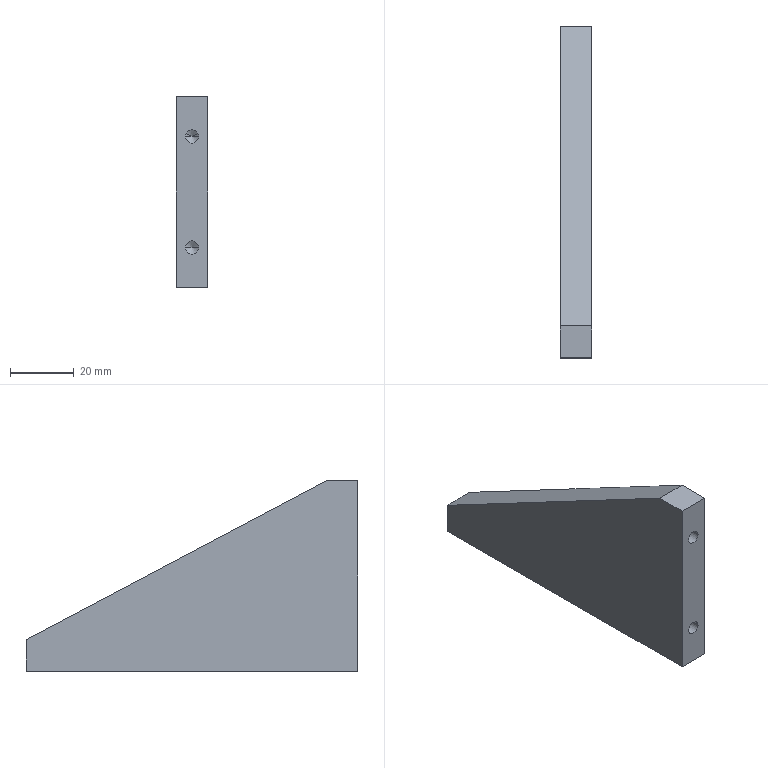Component | SolidWorks | 03-MilledRib-1 | 1 solid | 27 faces | box 10 x 104.5 x 60 mm | volume 38076 mm3 | cylinder 10 | cone 10 | plane 7 | commonest cylinder face diameters 4.2 x10
build123d program:
from build123d import *

# Parameters (mm, degrees)
EXTRUDE1_DEPTH        = 10
M5_TAPPED_HOLE1_D     = 4.2
M5_TAPPED_HOLE1_DEPTH = 14
M5_TAPPED_HOLE1_TIP   = 1.262
M5_TAPPED_HOLE2_D     = 4.2
M5_TAPPED_HOLE2_DEPTH = 14
M5_TAPPED_HOLE2_TIP   = 1.262


with BuildPart() as part:
    # Sketch1 → Extrude1 (new body)
    with BuildSketch(Plane.XY):
        Polygon((0, 0), (0, 104.5), (-10, 104.5), (-60, 10), (-60, 0), align=None)
    extrude(amount=EXTRUDE1_DEPTH)

    # M5 Tapped Hole1
    with Locations(Plane.XZ):
        with Locations((-47.5, 5), (-12.5, 5)):
            Hole(M5_TAPPED_HOLE1_D / 2, depth=M5_TAPPED_HOLE1_DEPTH)
            with Locations((0, 0, -(M5_TAPPED_HOLE1_DEPTH + M5_TAPPED_HOLE1_TIP / 2))):  # 118° drill point
                Cone(0, M5_TAPPED_HOLE1_D / 2, M5_TAPPED_HOLE1_TIP, mode=Mode.SUBTRACT)

    # M5 Tapped Hole2
    with Locations(Plane(origin=(0, 0, 0), x_dir=(0, 0, -1), z_dir=(1, 0, 0))):
        with Locations((-5, 89.5), (-5, 54.5), (-5, 19.5)):
            Hole(M5_TAPPED_HOLE2_D / 2, depth=M5_TAPPED_HOLE2_DEPTH)
            with Locations((0, 0, -(M5_TAPPED_HOLE2_DEPTH + M5_TAPPED_HOLE2_TIP / 2))):  # 118° drill point
                Cone(0, M5_TAPPED_HOLE2_D / 2, M5_TAPPED_HOLE2_TIP, mode=Mode.SUBTRACT)


solid = part.part

# Placed as in the assembly
solid = solid.moved(Location((-5, 56, -162.197), (0, 90, 0)))
STEP:
#1=CARTESIAN_POINT('',(0.08268,5.728,-5.835));
#2=VERTEX_POINT('',#1);
#3=CARTESIAN_POINT('',(-0.08268,5.728,-5.835));
#4=VERTEX_POINT('',#3);
#5=CARTESIAN_POINT('',(-0.,5.728,-5.835));
#6=DIRECTION('',(-0.,0.,-1.));
#7=DIRECTION('',(-1.,0.,0.));
#8=AXIS2_PLACEMENT_3D('',#5,#6,#7);
#9=CIRCLE('',#8,0.08268);
#10=EDGE_CURVE('',#2,#4,#9,.T.);
#11=ORIENTED_EDGE('',*,*,#10,.F.);
#12=CARTESIAN_POINT('',(0.08268,5.728,-6.386));
#13=VERTEX_POINT('',#12);
#14=CARTESIAN_POINT('',(0.08268,5.728,-6.386));
#15=DIRECTION('',(-0.,0.,-1.));
#16=VECTOR('',#15,39.37);
#17=LINE('',#14,#16);
#18=EDGE_CURVE('',#2,#13,#17,.T.);
#19=ORIENTED_EDGE('',*,*,#18,.T.);
#20=CARTESIAN_POINT('',(-0.08268,5.728,-6.386));
#21=VERTEX_POINT('',#20);
#22=CARTESIAN_POINT('',(-0.,5.728,-6.386));
#23=DIRECTION('',(-0.,0.,-1.));
#24=DIRECTION('',(-1.,0.,0.));
#25=AXIS2_PLACEMENT_3D('',#22,#23,#24);
#26=CIRCLE('',#25,0.08268);
#27=EDGE_CURVE('',#13,#21,#26,.T.);
#28=ORIENTED_EDGE('',*,*,#27,.T.);
#29=CARTESIAN_POINT('',(-0.08268,5.728,-6.386));
#30=DIRECTION('',(-0.,0.,-1.));
#31=VECTOR('',#30,39.37);
#32=LINE('',#29,#31);
#33=EDGE_CURVE('',#4,#21,#32,.T.);
#34=ORIENTED_EDGE('',*,*,#33,.F.);
#35=EDGE_LOOP('',(#11,#19,#28,#34));
#36=FACE_OUTER_BOUND('',#35,.T.);
#37=CARTESIAN_POINT('',(-0.,5.728,-6.386));
#38=DIRECTION('',(-0.,0.,-1.));
#39=DIRECTION('',(-1.,0.,0.));
#40=AXIS2_PLACEMENT_3D('',#37,#38,#39);
#41=CYLINDRICAL_SURFACE('',#40,0.08268);
#42=ADVANCED_FACE('',(#36),#41,.F.);
#43=CARTESIAN_POINT('',(-0.,5.728,-5.785));
#44=VERTEX_POINT('',#43);
#45=CARTESIAN_POINT('',(-0.08268,5.728,-5.835));
#46=DIRECTION('',(-0.8572,-0.,-0.515));
#47=VECTOR('',#46,39.37);
#48=LINE('',#45,#47);
#49=EDGE_CURVE('',#44,#4,#48,.T.);
#50=ORIENTED_EDGE('',*,*,#49,.F.);
#51=CARTESIAN_POINT('',(0.08268,5.728,-5.835));
#52=DIRECTION('',(0.8572,0.,-0.515));
#53=VECTOR('',#52,39.37);
#54=LINE('',#51,#53);
#55=EDGE_CURVE('',#44,#2,#54,.T.);
#56=ORIENTED_EDGE('',*,*,#55,.T.);
#57=ORIENTED_EDGE('',*,*,#10,.T.);
#58=EDGE_LOOP('',(#50,#56,#57));
#59=FACE_OUTER_BOUND('',#58,.T.);
#60=CARTESIAN_POINT('',(-0.,5.728,-5.835));
#61=DIRECTION('',(-0.,0.,-1.));
#62=DIRECTION('',(-1.,0.,0.));
#63=AXIS2_PLACEMENT_3D('',#60,#61,#62);
#64=CONICAL_SURFACE('',#63,0.08268,1.03);
#65=ADVANCED_FACE('',(#59),#64,.F.);
#66=CARTESIAN_POINT('',(0.08268,4.35,-5.835));
#67=VERTEX_POINT('',#66);
#68=CARTESIAN_POINT('',(-0.08268,4.35,-5.835));
#69=VERTEX_POINT('',#68);
#70=CARTESIAN_POINT('',(-0.,4.35,-5.835));
#71=DIRECTION('',(-0.,0.,-1.));
#72=DIRECTION('',(-1.,0.,0.));
#73=AXIS2_PLACEMENT_3D('',#70,#71,#72);
#74=CIRCLE('',#73,0.08268);
#75=EDGE_CURVE('',#67,#69,#74,.T.);
#76=ORIENTED_EDGE('',*,*,#75,.F.);
#77=CARTESIAN_POINT('',(0.08268,4.35,-6.386));
#78=VERTEX_POINT('',#77);
#79=CARTESIAN_POINT('',(0.08268,4.35,-6.386));
#80=DIRECTION('',(-0.,0.,-1.));
#81=VECTOR('',#80,39.37);
#82=LINE('',#79,#81);
#83=EDGE_CURVE('',#67,#78,#82,.T.);
#84=ORIENTED_EDGE('',*,*,#83,.T.);
#85=CARTESIAN_POINT('',(-0.08268,4.35,-6.386));
#86=VERTEX_POINT('',#85);
#87=CARTESIAN_POINT('',(-0.,4.35,-6.386));
#88=DIRECTION('',(-0.,0.,-1.));
#89=DIRECTION('',(-1.,0.,0.));
#90=AXIS2_PLACEMENT_3D('',#87,#88,#89);
#91=CIRCLE('',#90,0.08268);
#92=EDGE_CURVE('',#78,#86,#91,.T.);
#93=ORIENTED_EDGE('',*,*,#92,.T.);
#94=CARTESIAN_POINT('',(-0.08268,4.35,-6.386));
#95=DIRECTION('',(-0.,0.,-1.));
#96=VECTOR('',#95,39.37);
#97=LINE('',#94,#96);
#98=EDGE_CURVE('',#69,#86,#97,.T.);
#99=ORIENTED_EDGE('',*,*,#98,.F.);
#100=EDGE_LOOP('',(#76,#84,#93,#99));
#101=FACE_OUTER_BOUND('',#100,.T.);
#102=CARTESIAN_POINT('',(-0.,4.35,-6.386));
#103=DIRECTION('',(-0.,0.,-1.));
#104=DIRECTION('',(-1.,0.,0.));
#105=AXIS2_PLACEMENT_3D('',#102,#103,#104);
#106=CYLINDRICAL_SURFACE('',#105,0.08268);
#107=ADVANCED_FACE('',(#101),#106,.F.);
#108=CARTESIAN_POINT('',(-0.,4.35,-5.785));
#109=VERTEX_POINT('',#108);
#110=CARTESIAN_POINT('',(-0.08268,4.35,-5.835));
#111=DIRECTION('',(-0.8572,-0.,-0.515));
#112=VECTOR('',#111,39.37);
#113=LINE('',#110,#112);
#114=EDGE_CURVE('',#109,#69,#113,.T.);
#115=ORIENTED_EDGE('',*,*,#114,.F.);
#116=CARTESIAN_POINT('',(0.08268,4.35,-5.835));
#117=DIRECTION('',(0.8572,0.,-0.515));
#118=VECTOR('',#117,39.37);
#119=LINE('',#116,#118);
#120=EDGE_CURVE('',#109,#67,#119,.T.);
#121=ORIENTED_EDGE('',*,*,#120,.T.);
#122=ORIENTED_EDGE('',*,*,#75,.T.);
#123=EDGE_LOOP('',(#115,#121,#122));
#124=FACE_OUTER_BOUND('',#123,.T.);
#125=CARTESIAN_POINT('',(-0.,4.35,-5.835));
#126=DIRECTION('',(-0.,0.,-1.));
#127=DIRECTION('',(-1.,0.,0.));
#128=AXIS2_PLACEMENT_3D('',#125,#126,#127);
#129=CONICAL_SURFACE('',#128,0.08268,1.03);
#130=ADVANCED_FACE('',(#124),#129,.F.);
#131=CARTESIAN_POINT('',(0.08268,2.972,-5.835));
#132=VERTEX_POINT('',#131);
#133=CARTESIAN_POINT('',(-0.08268,2.972,-5.835));
#134=VERTEX_POINT('',#133);
#135=CARTESIAN_POINT('',(-0.,2.972,-5.835));
#136=DIRECTION('',(-0.,0.,-1.));
#137=DIRECTION('',(-1.,0.,0.));
#138=AXIS2_PLACEMENT_3D('',#135,#136,#137);
#139=CIRCLE('',#138,0.08268);
#140=EDGE_CURVE('',#132,#134,#139,.T.);
#141=ORIENTED_EDGE('',*,*,#140,.F.);
#142=CARTESIAN_POINT('',(0.08268,2.972,-6.386));
#143=VERTEX_POINT('',#142);
#144=CARTESIAN_POINT('',(0.08268,2.972,-6.386));
#145=DIRECTION('',(-0.,0.,-1.));
#146=VECTOR('',#145,39.37);
#147=LINE('',#144,#146);
#148=EDGE_CURVE('',#132,#143,#147,.T.);
#149=ORIENTED_EDGE('',*,*,#148,.T.);
#150=CARTESIAN_POINT('',(-0.08268,2.972,-6.386));
#151=VERTEX_POINT('',#150);
#152=CARTESIAN_POINT('',(-0.,2.972,-6.386));
#153=DIRECTION('',(-0.,0.,-1.));
#154=DIRECTION('',(-1.,0.,0.));
#155=AXIS2_PLACEMENT_3D('',#152,#153,#154);
#156=CIRCLE('',#155,0.08268);
#157=EDGE_CURVE('',#143,#151,#156,.T.);
#158=ORIENTED_EDGE('',*,*,#157,.T.);
#159=CARTESIAN_POINT('',(-0.08268,2.972,-6.386));
#160=DIRECTION('',(-0.,0.,-1.));
#161=VECTOR('',#160,39.37);
#162=LINE('',#159,#161);
#163=EDGE_CURVE('',#134,#151,#162,.T.);
#164=ORIENTED_EDGE('',*,*,#163,.F.);
#165=EDGE_LOOP('',(#141,#149,#158,#164));
#166=FACE_OUTER_BOUND('',#165,.T.);
#167=CARTESIAN_POINT('',(-0.,2.972,-6.386));
#168=DIRECTION('',(-0.,0.,-1.));
#169=DIRECTION('',(-1.,0.,0.));
#170=AXIS2_PLACEMENT_3D('',#167,#168,#169);
#171=CYLINDRICAL_SURFACE('',#170,0.08268);
#172=ADVANCED_FACE('',(#166),#171,.F.);
#173=CARTESIAN_POINT('',(-0.,2.972,-5.785));
#174=VERTEX_POINT('',#173);
#175=CARTESIAN_POINT('',(-0.08268,2.972,-5.835));
#176=DIRECTION('',(-0.8572,-0.,-0.515));
#177=VECTOR('',#176,39.37);
#178=LINE('',#175,#177);
#179=EDGE_CURVE('',#174,#134,#178,.T.);
#180=ORIENTED_EDGE('',*,*,#179,.F.);
#181=CARTESIAN_POINT('',(0.08268,2.972,-5.835));
#182=DIRECTION('',(0.8572,0.,-0.515));
#183=VECTOR('',#182,39.37);
#184=LINE('',#181,#183);
#185=EDGE_CURVE('',#174,#132,#184,.T.);
#186=ORIENTED_EDGE('',*,*,#185,.T.);
#187=ORIENTED_EDGE('',*,*,#140,.T.);
#188=EDGE_LOOP('',(#180,#186,#187));
#189=FACE_OUTER_BOUND('',#188,.T.);
#190=CARTESIAN_POINT('',(-0.,2.972,-5.835));
#191=DIRECTION('',(-0.,0.,-1.));
#192=DIRECTION('',(-1.,0.,0.));
#193=AXIS2_PLACEMENT_3D('',#190,#191,#192);
#194=CONICAL_SURFACE('',#193,0.08268,1.03);
#195=ADVANCED_FACE('',(#189),#194,.F.);
#196=CARTESIAN_POINT('',(0.08268,2.756,-4.516));
#197=VERTEX_POINT('',#196);
#198=CARTESIAN_POINT('',(-0.08268,2.756,-4.516));
#199=VERTEX_POINT('',#198);
#200=CARTESIAN_POINT('',(-0.,2.756,-4.516));
#201=DIRECTION('',(0.,-1.,-0.));
#202=DIRECTION('',(-1.,0.,0.));
#203=AXIS2_PLACEMENT_3D('',#200,#201,#202);
#204=CIRCLE('',#203,0.08268);
#205=EDGE_CURVE('',#197,#199,#204,.T.);
#206=ORIENTED_EDGE('',*,*,#205,.F.);
#207=CARTESIAN_POINT('',(0.08268,2.205,-4.516));
#208=VERTEX_POINT('',#207);
#209=CARTESIAN_POINT('',(0.08268,2.205,-4.516));
#210=DIRECTION('',(0.,-1.,-0.));
#211=VECTOR('',#210,39.37);
#212=LINE('',#209,#211);
#213=EDGE_CURVE('',#197,#208,#212,.T.);
#214=ORIENTED_EDGE('',*,*,#213,.T.);
#215=CARTESIAN_POINT('',(-0.08268,2.205,-4.516));
#216=VERTEX_POINT('',#215);
#217=CARTESIAN_POINT('',(-0.,2.205,-4.516));
#218=DIRECTION('',(0.,-1.,-0.));
#219=DIRECTION('',(-1.,0.,0.));
#220=AXIS2_PLACEMENT_3D('',#217,#218,#219);
#221=CIRCLE('',#220,0.08268);
#222=EDGE_CURVE('',#208,#216,#221,.T.);
#223=ORIENTED_EDGE('',*,*,#222,.T.);
#224=CARTESIAN_POINT('',(-0.08268,2.205,-4.516));
#225=DIRECTION('',(0.,-1.,-0.));
#226=VECTOR('',#225,39.37);
#227=LINE('',#224,#226);
#228=EDGE_CURVE('',#199,#216,#227,.T.);
#229=ORIENTED_EDGE('',*,*,#228,.F.);
#230=EDGE_LOOP('',(#206,#214,#223,#229));
#231=FACE_OUTER_BOUND('',#230,.T.);
#232=CARTESIAN_POINT('',(-0.,2.205,-4.516));
#233=DIRECTION('',(0.,-1.,-0.));
#234=DIRECTION('',(-1.,0.,0.));
#235=AXIS2_PLACEMENT_3D('',#232,#233,#234);
#236=CYLINDRICAL_SURFACE('',#235,0.08268);
#237=ADVANCED_FACE('',(#231),#236,.F.);
#238=CARTESIAN_POINT('',(-0.,2.806,-4.516));
#239=VERTEX_POINT('',#238);
#240=CARTESIAN_POINT('',(-0.08268,2.756,-4.516));
#241=DIRECTION('',(-0.8572,-0.515,0.));
#242=VECTOR('',#241,39.37);
#243=LINE('',#240,#242);
#244=EDGE_CURVE('',#239,#199,#243,.T.);
#245=ORIENTED_EDGE('',*,*,#244,.F.);
#246=CARTESIAN_POINT('',(0.08268,2.756,-4.516));
#247=DIRECTION('',(0.8572,-0.515,-0.));
#248=VECTOR('',#247,39.37);
#249=LINE('',#246,#248);
#250=EDGE_CURVE('',#239,#197,#249,.T.);
#251=ORIENTED_EDGE('',*,*,#250,.T.);
#252=ORIENTED_EDGE('',*,*,#205,.T.);
#253=EDGE_LOOP('',(#245,#251,#252));
#254=FACE_OUTER_BOUND('',#253,.T.);
#255=CARTESIAN_POINT('',(-0.,2.756,-4.516));
#256=DIRECTION('',(0.,-1.,-0.));
#257=DIRECTION('',(-1.,0.,0.));
#258=AXIS2_PLACEMENT_3D('',#255,#256,#257);
#259=CONICAL_SURFACE('',#258,0.08268,1.03);
#260=ADVANCED_FACE('',(#254),#259,.F.);
#261=CARTESIAN_POINT('',(0.08268,2.756,-5.894));
#262=VERTEX_POINT('',#261);
#263=CARTESIAN_POINT('',(-0.08268,2.756,-5.894));
#264=VERTEX_POINT('',#263);
#265=CARTESIAN_POINT('',(-0.,2.756,-5.894));
#266=DIRECTION('',(0.,-1.,-0.));
#267=DIRECTION('',(-1.,0.,0.));
#268=AXIS2_PLACEMENT_3D('',#265,#266,#267);
#269=CIRCLE('',#268,0.08268);
#270=EDGE_CURVE('',#262,#264,#269,.T.);
#271=ORIENTED_EDGE('',*,*,#270,.F.);
#272=CARTESIAN_POINT('',(0.08268,2.205,-5.894));
#273=VERTEX_POINT('',#272);
#274=CARTESIAN_POINT('',(0.08268,2.205,-5.894));
#275=DIRECTION('',(0.,-1.,-0.));
#276=VECTOR('',#275,39.37);
#277=LINE('',#274,#276);
#278=EDGE_CURVE('',#262,#273,#277,.T.);
#279=ORIENTED_EDGE('',*,*,#278,.T.);
#280=CARTESIAN_POINT('',(-0.08268,2.205,-5.894));
#281=VERTEX_POINT('',#280);
#282=CARTESIAN_POINT('',(-0.,2.205,-5.894));
#283=DIRECTION('',(0.,-1.,-0.));
#284=DIRECTION('',(-1.,0.,0.));
#285=AXIS2_PLACEMENT_3D('',#282,#283,#284);
#286=CIRCLE('',#285,0.08268);
#287=EDGE_CURVE('',#273,#281,#286,.T.);
#288=ORIENTED_EDGE('',*,*,#287,.T.);
#289=CARTESIAN_POINT('',(-0.08268,2.205,-5.894));
#290=DIRECTION('',(0.,-1.,-0.));
#291=VECTOR('',#290,39.37);
#292=LINE('',#289,#291);
#293=EDGE_CURVE('',#264,#281,#292,.T.);
#294=ORIENTED_EDGE('',*,*,#293,.F.);
#295=EDGE_LOOP('',(#271,#279,#288,#294));
#296=FACE_OUTER_BOUND('',#295,.T.);
#297=CARTESIAN_POINT('',(-0.,2.205,-5.894));
#298=DIRECTION('',(0.,-1.,-0.));
#299=DIRECTION('',(-1.,0.,0.));
#300=AXIS2_PLACEMENT_3D('',#297,#298,#299);
#301=CYLINDRICAL_SURFACE('',#300,0.08268);
#302=ADVANCED_FACE('',(#296),#301,.F.);
#303=CARTESIAN_POINT('',(-0.,2.806,-5.894));
#304=VERTEX_POINT('',#303);
#305=CARTESIAN_POINT('',(-0.08268,2.756,-5.894));
#306=DIRECTION('',(-0.8572,-0.515,0.));
#307=VECTOR('',#306,39.37);
#308=LINE('',#305,#307);
#309=EDGE_CURVE('',#304,#264,#308,.T.);
#310=ORIENTED_EDGE('',*,*,#309,.F.);
#311=CARTESIAN_POINT('',(0.08268,2.756,-5.894));
#312=DIRECTION('',(0.8572,-0.515,-0.));
#313=VECTOR('',#312,39.37);
#314=LINE('',#311,#313);
#315=EDGE_CURVE('',#304,#262,#314,.T.);
#316=ORIENTED_EDGE('',*,*,#315,.T.);
#317=ORIENTED_EDGE('',*,*,#270,.T.);
#318=EDGE_LOOP('',(#310,#316,#317));
#319=FACE_OUTER_BOUND('',#318,.T.);
#320=CARTESIAN_POINT('',(-0.,2.756,-5.894));
#321=DIRECTION('',(0.,-1.,-0.));
#322=DIRECTION('',(-1.,0.,0.));
#323=AXIS2_PLACEMENT_3D('',#320,#321,#322);
#324=CONICAL_SURFACE('',#323,0.08268,1.03);
#325=ADVANCED_FACE('',(#319),#324,.F.);
#326=CARTESIAN_POINT('',(-0.,2.205,-4.516));
#327=DIRECTION('',(0.,-1.,-0.));
#328=DIRECTION('',(-1.,0.,0.));
#329=AXIS2_PLACEMENT_3D('',#326,#327,#328);
#330=CIRCLE('',#329,0.08268);
#331=EDGE_CURVE('',#216,#208,#330,.T.);
#332=ORIENTED_EDGE('',*,*,#331,.F.);
#333=ORIENTED_EDGE('',*,*,#222,.F.);
#334=EDGE_LOOP('',(#332,#333));
#335=FACE_BOUND('',#334,.T.);
#336=CARTESIAN_POINT('',(-0.,2.205,-5.894));
#337=DIRECTION('',(0.,-1.,-0.));
#338=DIRECTION('',(-1.,0.,0.));
#339=AXIS2_PLACEMENT_3D('',#336,#337,#338);
#340=CIRCLE('',#339,0.08268);
#341=EDGE_CURVE('',#281,#273,#340,.T.);
#342=ORIENTED_EDGE('',*,*,#341,.F.);
#343=ORIENTED_EDGE('',*,*,#287,.F.);
#344=EDGE_LOOP('',(#342,#343));
#345=FACE_BOUND('',#344,.T.);
#346=CARTESIAN_POINT('',(-0.1969,2.205,-4.024));
#347=VERTEX_POINT('',#346);
#348=CARTESIAN_POINT('',(-0.1969,2.205,-6.386));
#349=VERTEX_POINT('',#348);
#350=CARTESIAN_POINT('',(-0.1969,2.205,-4.024));
#351=DIRECTION('',(-0.,0.,-1.));
#352=VECTOR('',#351,39.37);
#353=LINE('',#350,#352);
#354=EDGE_CURVE('',#347,#349,#353,.T.);
#355=ORIENTED_EDGE('',*,*,#354,.T.);
#356=CARTESIAN_POINT('',(0.1969,2.205,-6.386));
#357=VERTEX_POINT('',#356);
#358=CARTESIAN_POINT('',(0.1969,2.205,-6.386));
#359=DIRECTION('',(-1.,-0.,0.));
#360=VECTOR('',#359,39.37);
#361=LINE('',#358,#360);
#362=EDGE_CURVE('',#357,#349,#361,.T.);
#363=ORIENTED_EDGE('',*,*,#362,.F.);
#364=CARTESIAN_POINT('',(0.1969,2.205,-4.024));
#365=VERTEX_POINT('',#364);
#366=CARTESIAN_POINT('',(0.1969,2.205,-4.024));
#367=DIRECTION('',(-0.,0.,-1.));
#368=VECTOR('',#367,39.37);
#369=LINE('',#366,#368);
#370=EDGE_CURVE('',#365,#357,#369,.T.);
#371=ORIENTED_EDGE('',*,*,#370,.F.);
#372=CARTESIAN_POINT('',(0.1969,2.205,-4.024));
#373=DIRECTION('',(-1.,-0.,0.));
#374=VECTOR('',#373,39.37);
#375=LINE('',#372,#374);
#376=EDGE_CURVE('',#365,#347,#375,.T.);
#377=ORIENTED_EDGE('',*,*,#376,.T.);
#378=EDGE_LOOP('',(#355,#363,#371,#377));
#379=FACE_OUTER_BOUND('',#378,.T.);
#380=CARTESIAN_POINT('',(0.1969,2.205,-4.024));
#381=DIRECTION('',(-0.,1.,0.));
#382=DIRECTION('',(1.,0.,-0.));
#383=AXIS2_PLACEMENT_3D('',#380,#381,#382);
#384=PLANE('',#383);
#385=ADVANCED_FACE('',(#335,#345,#379),#384,.F.);
#386=CARTESIAN_POINT('',(-0.,5.728,-6.386));
#387=DIRECTION('',(-0.,0.,-1.));
#388=DIRECTION('',(-1.,0.,0.));
#389=AXIS2_PLACEMENT_3D('',#386,#387,#388);
#390=CIRCLE('',#389,0.08268);
#391=EDGE_CURVE('',#21,#13,#390,.T.);
#392=ORIENTED_EDGE('',*,*,#391,.F.);
#393=ORIENTED_EDGE('',*,*,#27,.F.);
#394=EDGE_LOOP('',(#392,#393));
#395=FACE_BOUND('',#394,.T.);
#396=CARTESIAN_POINT('',(-0.,4.35,-6.386));
#397=DIRECTION('',(-0.,0.,-1.));
#398=DIRECTION('',(-1.,0.,0.));
#399=AXIS2_PLACEMENT_3D('',#396,#397,#398);
#400=CIRCLE('',#399,0.08268);
#401=EDGE_CURVE('',#86,#78,#400,.T.);
#402=ORIENTED_EDGE('',*,*,#401,.F.);
#403=ORIENTED_EDGE('',*,*,#92,.F.);
#404=EDGE_LOOP('',(#402,#403));
#405=FACE_BOUND('',#404,.T.);
#406=CARTESIAN_POINT('',(-0.,2.972,-6.386));
#407=DIRECTION('',(-0.,0.,-1.));
#408=DIRECTION('',(-1.,0.,0.));
#409=AXIS2_PLACEMENT_3D('',#406,#407,#408);
#410=CIRCLE('',#409,0.08268);
#411=EDGE_CURVE('',#151,#143,#410,.T.);
#412=ORIENTED_EDGE('',*,*,#411,.F.);
#413=ORIENTED_EDGE('',*,*,#157,.F.);
#414=EDGE_LOOP('',(#412,#413));
#415=FACE_BOUND('',#414,.T.);
#416=CARTESIAN_POINT('',(-0.1969,6.319,-6.386));
#417=VERTEX_POINT('',#416);
#418=CARTESIAN_POINT('',(-0.1969,2.205,-6.386));
#419=DIRECTION('',(-0.,1.,0.));
#420=VECTOR('',#419,39.37);
#421=LINE('',#418,#420);
#422=EDGE_CURVE('',#349,#417,#421,.T.);
#423=ORIENTED_EDGE('',*,*,#422,.T.);
#424=CARTESIAN_POINT('',(0.1969,6.319,-6.386));
#425=VERTEX_POINT('',#424);
#426=CARTESIAN_POINT('',(0.1969,6.319,-6.386));
#427=DIRECTION('',(-1.,-0.,0.));
#428=VECTOR('',#427,39.37);
#429=LINE('',#426,#428);
#430=EDGE_CURVE('',#425,#417,#429,.T.);
#431=ORIENTED_EDGE('',*,*,#430,.F.);
#432=CARTESIAN_POINT('',(0.1969,2.205,-6.386));
#433=DIRECTION('',(-0.,1.,0.));
#434=VECTOR('',#433,39.37);
#435=LINE('',#432,#434);
#436=EDGE_CURVE('',#357,#425,#435,.T.);
#437=ORIENTED_EDGE('',*,*,#436,.F.);
#438=ORIENTED_EDGE('',*,*,#362,.T.);
#439=EDGE_LOOP('',(#423,#431,#437,#438));
#440=FACE_OUTER_BOUND('',#439,.T.);
#441=CARTESIAN_POINT('',(0.1969,2.205,-6.386));
#442=DIRECTION('',(0.,-0.,1.));
#443=DIRECTION('',(1.,0.,-0.));
#444=AXIS2_PLACEMENT_3D('',#441,#442,#443);
#445=PLANE('',#444);
#446=ADVANCED_FACE('',(#395,#405,#415,#440),#445,.F.);
#447=CARTESIAN_POINT('',(-0.1969,6.319,-5.992));
#448=VERTEX_POINT('',#447);
#449=CARTESIAN_POINT('',(-0.1969,6.319,-6.386));
#450=DIRECTION('',(0.,-0.,1.));
#451=VECTOR('',#450,39.37);
#452=LINE('',#449,#451);
#453=EDGE_CURVE('',#417,#448,#452,.T.);
#454=ORIENTED_EDGE('',*,*,#453,.T.);
#455=CARTESIAN_POINT('',(0.1969,6.319,-5.992));
#456=VERTEX_POINT('',#455);
#457=CARTESIAN_POINT('',(0.1969,6.319,-5.992));
#458=DIRECTION('',(-1.,-0.,0.));
#459=VECTOR('',#458,39.37);
#460=LINE('',#457,#459);
#461=EDGE_CURVE('',#456,#448,#460,.T.);
#462=ORIENTED_EDGE('',*,*,#461,.F.);
#463=CARTESIAN_POINT('',(0.1969,6.319,-6.386));
#464=DIRECTION('',(0.,-0.,1.));
#465=VECTOR('',#464,39.37);
#466=LINE('',#463,#465);
#467=EDGE_CURVE('',#425,#456,#466,.T.);
#468=ORIENTED_EDGE('',*,*,#467,.F.);
#469=ORIENTED_EDGE('',*,*,#430,.T.);
#470=EDGE_LOOP('',(#454,#462,#468,#469));
#471=FACE_OUTER_BOUND('',#470,.T.);
#472=CARTESIAN_POINT('',(0.1969,6.319,-6.386));
#473=DIRECTION('',(0.,-1.,-0.));
#474=DIRECTION('',(-1.,-0.,0.));
#475=AXIS2_PLACEMENT_3D('',#472,#473,#474);
#476=PLANE('',#475);
#477=ADVANCED_FACE('',(#471),#476,.F.);
#478=CARTESIAN_POINT('',(-0.1969,2.598,-4.024));
#479=VERTEX_POINT('',#478);
#480=CARTESIAN_POINT('',(-0.1969,6.319,-5.992));
#481=DIRECTION('',(0.,-0.8839,0.4677));
#482=VECTOR('',#481,39.37);
#483=LINE('',#480,#482);
#484=EDGE_CURVE('',#448,#479,#483,.T.);
#485=ORIENTED_EDGE('',*,*,#484,.T.);
#486=CARTESIAN_POINT('',(0.1969,2.598,-4.024));
#487=VERTEX_POINT('',#486);
#488=CARTESIAN_POINT('',(0.1969,2.598,-4.024));
#489=DIRECTION('',(-1.,-0.,0.));
#490=VECTOR('',#489,39.37);
#491=LINE('',#488,#490);
#492=EDGE_CURVE('',#487,#479,#491,.T.);
#493=ORIENTED_EDGE('',*,*,#492,.F.);
#494=CARTESIAN_POINT('',(0.1969,6.319,-5.992));
#495=DIRECTION('',(0.,-0.8839,0.4677));
#496=VECTOR('',#495,39.37);
#497=LINE('',#494,#496);
#498=EDGE_CURVE('',#456,#487,#497,.T.);
#499=ORIENTED_EDGE('',*,*,#498,.F.);
#500=ORIENTED_EDGE('',*,*,#461,.T.);
#501=EDGE_LOOP('',(#485,#493,#499,#500));
#502=FACE_OUTER_BOUND('',#501,.T.);
#503=CARTESIAN_POINT('',(0.1969,6.319,-5.992));
#504=DIRECTION('',(-0.,-0.4677,-0.8839));
#505=DIRECTION('',(-0.,0.8839,-0.4677));
#506=AXIS2_PLACEMENT_3D('',#503,#504,#505);
#507=PLANE('',#506);
#508=ADVANCED_FACE('',(#502),#507,.F.);
#509=CARTESIAN_POINT('',(-0.1969,2.598,-4.024));
#510=DIRECTION('',(0.,-1.,-0.));
#511=VECTOR('',#510,39.37);
#512=LINE('',#509,#511);
#513=EDGE_CURVE('',#479,#347,#512,.T.);
#514=ORIENTED_EDGE('',*,*,#513,.T.);
#515=ORIENTED_EDGE('',*,*,#376,.F.);
#516=CARTESIAN_POINT('',(0.1969,2.598,-4.024));
#517=DIRECTION('',(0.,-1.,-0.));
#518=VECTOR('',#517,39.37);
#519=LINE('',#516,#518);
#520=EDGE_CURVE('',#487,#365,#519,.T.);
#521=ORIENTED_EDGE('',*,*,#520,.F.);
#522=ORIENTED_EDGE('',*,*,#492,.T.);
#523=EDGE_LOOP('',(#514,#515,#521,#522));
#524=FACE_OUTER_BOUND('',#523,.T.);
#525=CARTESIAN_POINT('',(0.1969,2.598,-4.024));
#526=DIRECTION('',(-0.,0.,-1.));
#527=DIRECTION('',(-1.,-0.,0.));
#528=AXIS2_PLACEMENT_3D('',#525,#526,#527);
#529=PLANE('',#528);
#530=ADVANCED_FACE('',(#524),#529,.F.);
#531=ORIENTED_EDGE('',*,*,#370,.T.);
#532=ORIENTED_EDGE('',*,*,#436,.T.);
#533=ORIENTED_EDGE('',*,*,#467,.T.);
#534=ORIENTED_EDGE('',*,*,#498,.T.);
#535=ORIENTED_EDGE('',*,*,#520,.T.);
#536=EDGE_LOOP('',(#531,#532,#533,#534,#535));
#537=FACE_OUTER_BOUND('',#536,.T.);
#538=CARTESIAN_POINT('',(0.1969,2.205,-6.386));
#539=DIRECTION('',(1.,0.,-0.));
#540=DIRECTION('',(-0.,0.,-1.));
#541=AXIS2_PLACEMENT_3D('',#538,#539,#540);
#542=PLANE('',#541);
#543=ADVANCED_FACE('',(#537),#542,.T.);
#544=ORIENTED_EDGE('',*,*,#354,.F.);
#545=ORIENTED_EDGE('',*,*,#513,.F.);
#546=ORIENTED_EDGE('',*,*,#484,.F.);
#547=ORIENTED_EDGE('',*,*,#453,.F.);
#548=ORIENTED_EDGE('',*,*,#422,.F.);
#549=EDGE_LOOP('',(#544,#545,#546,#547,#548));
#550=FACE_OUTER_BOUND('',#549,.T.);
#551=CARTESIAN_POINT('',(-0.1969,2.205,-6.386));
#552=DIRECTION('',(1.,0.,-0.));
#553=DIRECTION('',(-0.,0.,-1.));
#554=AXIS2_PLACEMENT_3D('',#551,#552,#553);
#555=PLANE('',#554);
#556=ADVANCED_FACE('',(#550),#555,.F.);
#557=ORIENTED_EDGE('',*,*,#315,.F.);
#558=ORIENTED_EDGE('',*,*,#309,.T.);
#559=CARTESIAN_POINT('',(-0.,2.756,-5.894));
#560=DIRECTION('',(0.,-1.,-0.));
#561=DIRECTION('',(-1.,0.,0.));
#562=AXIS2_PLACEMENT_3D('',#559,#560,#561);
#563=CIRCLE('',#562,0.08268);
#564=EDGE_CURVE('',#264,#262,#563,.T.);
#565=ORIENTED_EDGE('',*,*,#564,.T.);
#566=EDGE_LOOP('',(#557,#558,#565));
#567=FACE_OUTER_BOUND('',#566,.T.);
#568=CARTESIAN_POINT('',(-0.,2.756,-5.894));
#569=DIRECTION('',(0.,-1.,-0.));
#570=DIRECTION('',(-1.,0.,0.));
#571=AXIS2_PLACEMENT_3D('',#568,#569,#570);
#572=CONICAL_SURFACE('',#571,0.08268,1.03);
#573=ADVANCED_FACE('',(#567),#572,.F.);
#574=ORIENTED_EDGE('',*,*,#278,.F.);
#575=ORIENTED_EDGE('',*,*,#564,.F.);
#576=ORIENTED_EDGE('',*,*,#293,.T.);
#577=ORIENTED_EDGE('',*,*,#341,.T.);
#578=EDGE_LOOP('',(#574,#575,#576,#577));
#579=FACE_OUTER_BOUND('',#578,.T.);
#580=CARTESIAN_POINT('',(-0.,2.205,-5.894));
#581=DIRECTION('',(0.,-1.,-0.));
#582=DIRECTION('',(-1.,0.,0.));
#583=AXIS2_PLACEMENT_3D('',#580,#581,#582);
#584=CYLINDRICAL_SURFACE('',#583,0.08268);
#585=ADVANCED_FACE('',(#579),#584,.F.);
#586=ORIENTED_EDGE('',*,*,#250,.F.);
#587=ORIENTED_EDGE('',*,*,#244,.T.);
#588=CARTESIAN_POINT('',(-0.,2.756,-4.516));
#589=DIRECTION('',(0.,-1.,-0.));
#590=DIRECTION('',(-1.,0.,0.));
#591=AXIS2_PLACEMENT_3D('',#588,#589,#590);
#592=CIRCLE('',#591,0.08268);
#593=EDGE_CURVE('',#199,#197,#592,.T.);
#594=ORIENTED_EDGE('',*,*,#593,.T.);
#595=EDGE_LOOP('',(#586,#587,#594));
#596=FACE_OUTER_BOUND('',#595,.T.);
#597=CARTESIAN_POINT('',(-0.,2.756,-4.516));
#598=DIRECTION('',(0.,-1.,-0.));
#599=DIRECTION('',(-1.,0.,0.));
#600=AXIS2_PLACEMENT_3D('',#597,#598,#599);
#601=CONICAL_SURFACE('',#600,0.08268,1.03);
#602=ADVANCED_FACE('',(#596),#601,.F.);
#603=ORIENTED_EDGE('',*,*,#213,.F.);
#604=ORIENTED_EDGE('',*,*,#593,.F.);
#605=ORIENTED_EDGE('',*,*,#228,.T.);
#606=ORIENTED_EDGE('',*,*,#331,.T.);
#607=EDGE_LOOP('',(#603,#604,#605,#606));
#608=FACE_OUTER_BOUND('',#607,.T.);
#609=CARTESIAN_POINT('',(-0.,2.205,-4.516));
#610=DIRECTION('',(0.,-1.,-0.));
#611=DIRECTION('',(-1.,0.,0.));
#612=AXIS2_PLACEMENT_3D('',#609,#610,#611);
#613=CYLINDRICAL_SURFACE('',#612,0.08268);
#614=ADVANCED_FACE('',(#608),#613,.F.);
#615=ORIENTED_EDGE('',*,*,#185,.F.);
#616=ORIENTED_EDGE('',*,*,#179,.T.);
#617=CARTESIAN_POINT('',(-0.,2.972,-5.835));
#618=DIRECTION('',(-0.,0.,-1.));
#619=DIRECTION('',(-1.,0.,0.));
#620=AXIS2_PLACEMENT_3D('',#617,#618,#619);
#621=CIRCLE('',#620,0.08268);
#622=EDGE_CURVE('',#134,#132,#621,.T.);
#623=ORIENTED_EDGE('',*,*,#622,.T.);
#624=EDGE_LOOP('',(#615,#616,#623));
#625=FACE_OUTER_BOUND('',#624,.T.);
#626=CARTESIAN_POINT('',(-0.,2.972,-5.835));
#627=DIRECTION('',(-0.,0.,-1.));
#628=DIRECTION('',(-1.,0.,0.));
#629=AXIS2_PLACEMENT_3D('',#626,#627,#628);
#630=CONICAL_SURFACE('',#629,0.08268,1.03);
#631=ADVANCED_FACE('',(#625),#630,.F.);
#632=ORIENTED_EDGE('',*,*,#148,.F.);
#633=ORIENTED_EDGE('',*,*,#622,.F.);
#634=ORIENTED_EDGE('',*,*,#163,.T.);
#635=ORIENTED_EDGE('',*,*,#411,.T.);
#636=EDGE_LOOP('',(#632,#633,#634,#635));
#637=FACE_OUTER_BOUND('',#636,.T.);
#638=CARTESIAN_POINT('',(-0.,2.972,-6.386));
#639=DIRECTION('',(-0.,0.,-1.));
#640=DIRECTION('',(-1.,0.,0.));
#641=AXIS2_PLACEMENT_3D('',#638,#639,#640);
#642=CYLINDRICAL_SURFACE('',#641,0.08268);
#643=ADVANCED_FACE('',(#637),#642,.F.);
#644=ORIENTED_EDGE('',*,*,#120,.F.);
#645=ORIENTED_EDGE('',*,*,#114,.T.);
#646=CARTESIAN_POINT('',(-0.,4.35,-5.835));
#647=DIRECTION('',(-0.,0.,-1.));
#648=DIRECTION('',(-1.,0.,0.));
#649=AXIS2_PLACEMENT_3D('',#646,#647,#648);
#650=CIRCLE('',#649,0.08268);
#651=EDGE_CURVE('',#69,#67,#650,.T.);
#652=ORIENTED_EDGE('',*,*,#651,.T.);
#653=EDGE_LOOP('',(#644,#645,#652));
#654=FACE_OUTER_BOUND('',#653,.T.);
#655=CARTESIAN_POINT('',(-0.,4.35,-5.835));
#656=DIRECTION('',(-0.,0.,-1.));
#657=DIRECTION('',(-1.,0.,0.));
#658=AXIS2_PLACEMENT_3D('',#655,#656,#657);
#659=CONICAL_SURFACE('',#658,0.08268,1.03);
#660=ADVANCED_FACE('',(#654),#659,.F.);
#661=ORIENTED_EDGE('',*,*,#83,.F.);
#662=ORIENTED_EDGE('',*,*,#651,.F.);
#663=ORIENTED_EDGE('',*,*,#98,.T.);
#664=ORIENTED_EDGE('',*,*,#401,.T.);
#665=EDGE_LOOP('',(#661,#662,#663,#664));
#666=FACE_OUTER_BOUND('',#665,.T.);
#667=CARTESIAN_POINT('',(-0.,4.35,-6.386));
#668=DIRECTION('',(-0.,0.,-1.));
#669=DIRECTION('',(-1.,0.,0.));
#670=AXIS2_PLACEMENT_3D('',#667,#668,#669);
#671=CYLINDRICAL_SURFACE('',#670,0.08268);
#672=ADVANCED_FACE('',(#666),#671,.F.);
#673=ORIENTED_EDGE('',*,*,#55,.F.);
#674=ORIENTED_EDGE('',*,*,#49,.T.);
#675=CARTESIAN_POINT('',(-0.,5.728,-5.835));
#676=DIRECTION('',(-0.,0.,-1.));
#677=DIRECTION('',(-1.,0.,0.));
#678=AXIS2_PLACEMENT_3D('',#675,#676,#677);
#679=CIRCLE('',#678,0.08268);
#680=EDGE_CURVE('',#4,#2,#679,.T.);
#681=ORIENTED_EDGE('',*,*,#680,.T.);
#682=EDGE_LOOP('',(#673,#674,#681));
#683=FACE_OUTER_BOUND('',#682,.T.);
#684=CARTESIAN_POINT('',(-0.,5.728,-5.835));
#685=DIRECTION('',(-0.,0.,-1.));
#686=DIRECTION('',(-1.,0.,0.));
#687=AXIS2_PLACEMENT_3D('',#684,#685,#686);
#688=CONICAL_SURFACE('',#687,0.08268,1.03);
#689=ADVANCED_FACE('',(#683),#688,.F.);
#690=ORIENTED_EDGE('',*,*,#18,.F.);
#691=ORIENTED_EDGE('',*,*,#680,.F.);
#692=ORIENTED_EDGE('',*,*,#33,.T.);
#693=ORIENTED_EDGE('',*,*,#391,.T.);
#694=EDGE_LOOP('',(#690,#691,#692,#693));
#695=FACE_OUTER_BOUND('',#694,.T.);
#696=CARTESIAN_POINT('',(-0.,5.728,-6.386));
#697=DIRECTION('',(-0.,0.,-1.));
#698=DIRECTION('',(-1.,0.,0.));
#699=AXIS2_PLACEMENT_3D('',#696,#697,#698);
#700=CYLINDRICAL_SURFACE('',#699,0.08268);
#701=ADVANCED_FACE('',(#695),#700,.F.);
#702=CLOSED_SHELL('',(#42,#65,#107,#130,#172,#195,#237,#260,#302,#325,#385,#446,#477,#508,#530,#543,#556,#573,#585,#602,#614,#631,#643,#660,#672,#689,#701));
#703=MANIFOLD_SOLID_BREP('',#702);
#704=CARTESIAN_POINT('',(0.,0.,0.));
#705=DIRECTION('',(0.,0.,1.));
#706=DIRECTION('',(1.,0.,0.));
#707=AXIS2_PLACEMENT_3D('',#704,#705,#706);
#708=(LENGTH_UNIT()NAMED_UNIT(*)SI_UNIT($,.METRE.));
#709=LENGTH_MEASURE_WITH_UNIT(LENGTH_MEASURE(0.0254),#708);
#710=DIMENSIONAL_EXPONENTS(1.,0.,0.,0.,0.,0.,0.);
#711=(CONVERSION_BASED_UNIT('',#709)LENGTH_UNIT()NAMED_UNIT(#710));
#712=UNCERTAINTY_MEASURE_WITH_UNIT(LENGTH_MEASURE(0.00001),#711,'','');
#713=(NAMED_UNIT(*)PLANE_ANGLE_UNIT()SI_UNIT($,.RADIAN.));
#714=(NAMED_UNIT(*)SI_UNIT($,.STERADIAN.)SOLID_ANGLE_UNIT());
#715=(GEOMETRIC_REPRESENTATION_CONTEXT(3)GLOBAL_UNCERTAINTY_ASSIGNED_CONTEXT((#712))GLOBAL_UNIT_ASSIGNED_CONTEXT((#711,#713,#714))REPRESENTATION_CONTEXT('',''));
#716=ADVANCED_BREP_SHAPE_REPRESENTATION('',(#703,#707),#715);
#717=COLOUR_RGB('',0.7922,0.8196,0.9333);
#718=FILL_AREA_STYLE_COLOUR('',#717);
#719=FILL_AREA_STYLE('',(#718));
#720=SURFACE_STYLE_FILL_AREA(#719);
#721=SURFACE_SIDE_STYLE('',(#720));
#722=SURFACE_STYLE_USAGE(.BOTH.,#721);
#723=PRESENTATION_STYLE_ASSIGNMENT((#722));
#724=STYLED_ITEM('',(#723),#703);
#725=(LENGTH_UNIT()NAMED_UNIT(*)SI_UNIT($,.METRE.));
#726=LENGTH_MEASURE_WITH_UNIT(LENGTH_MEASURE(0.0254),#725);
#727=DIMENSIONAL_EXPONENTS(1.,0.,0.,0.,0.,0.,0.);
#728=(CONVERSION_BASED_UNIT('',#726)LENGTH_UNIT()NAMED_UNIT(#727));
#729=UNCERTAINTY_MEASURE_WITH_UNIT(LENGTH_MEASURE(0.00001),#728,'','');
#730=(NAMED_UNIT(*)PLANE_ANGLE_UNIT()SI_UNIT($,.RADIAN.));
#731=(NAMED_UNIT(*)SI_UNIT($,.STERADIAN.)SOLID_ANGLE_UNIT());
#732=(GEOMETRIC_REPRESENTATION_CONTEXT(3)GLOBAL_UNCERTAINTY_ASSIGNED_CONTEXT((#729))GLOBAL_UNIT_ASSIGNED_CONTEXT((#728,#730,#731))REPRESENTATION_CONTEXT('',''));
#733=MECHANICAL_DESIGN_GEOMETRIC_PRESENTATION_REPRESENTATION('',(#724),#732);
#734=PRESENTATION_LAYER_ASSIGNMENT('','',(#724));